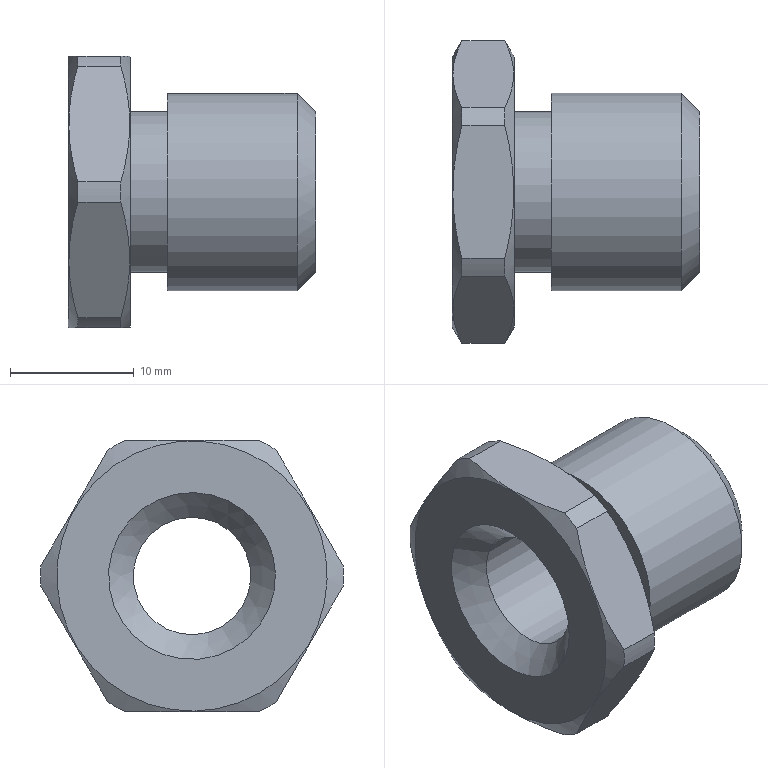Component | NX | INLET_SCREW | 1 solid | 23 faces | volume 3334 mm3 | plane 10 | cylinder 9 | cone 4 | commonest cylinder face diameters 24.5 x6 16 x1 13 x1 9.5 x1